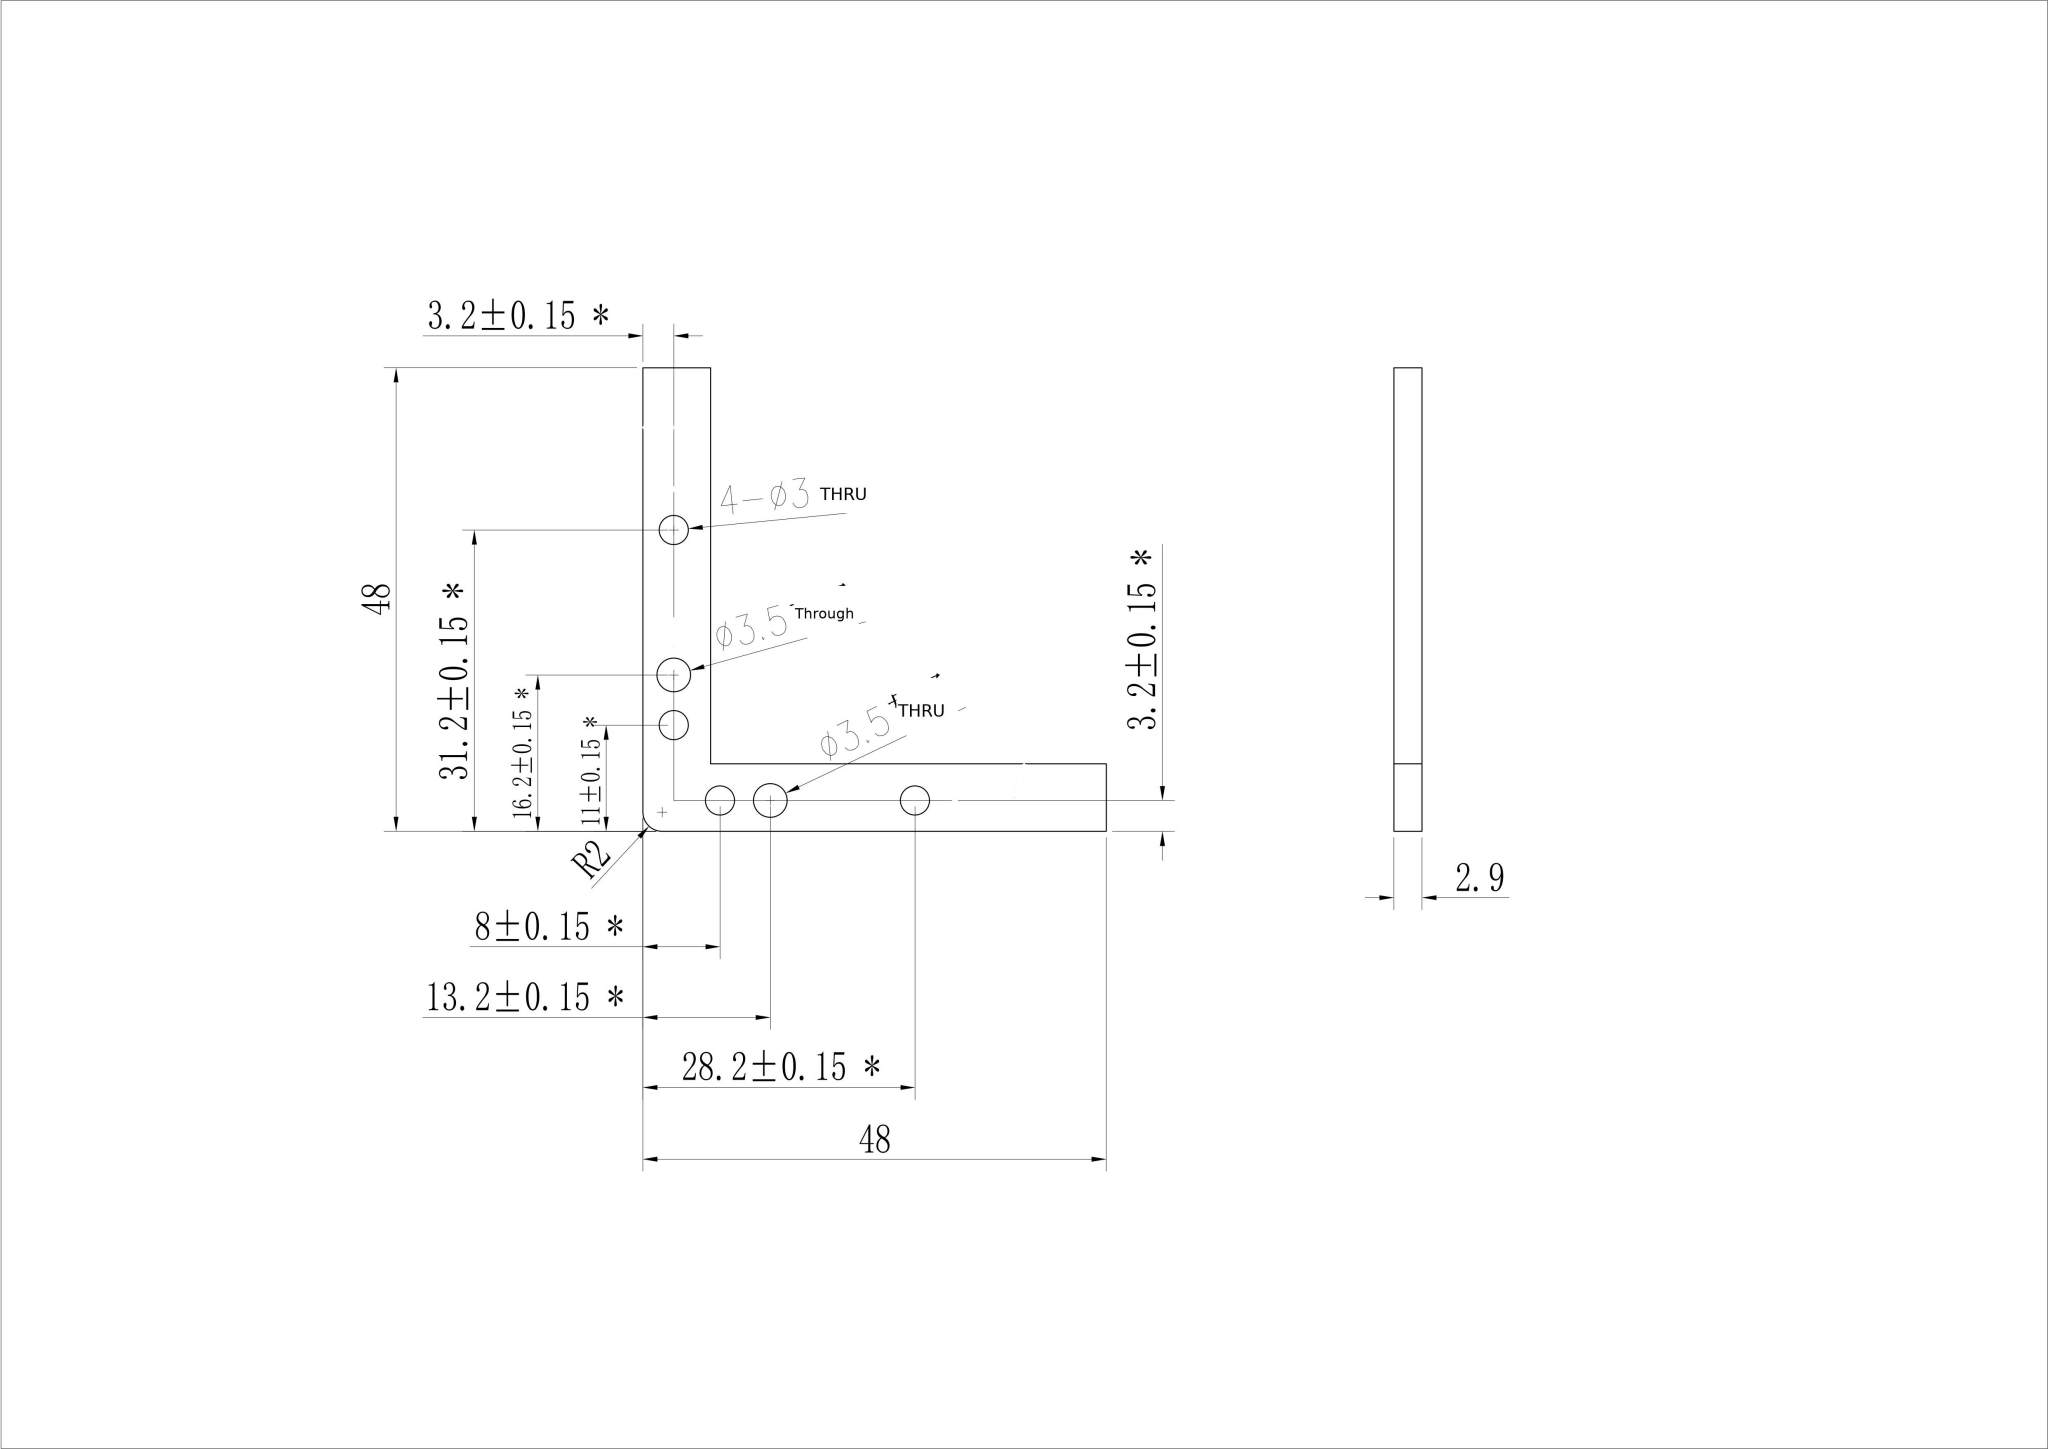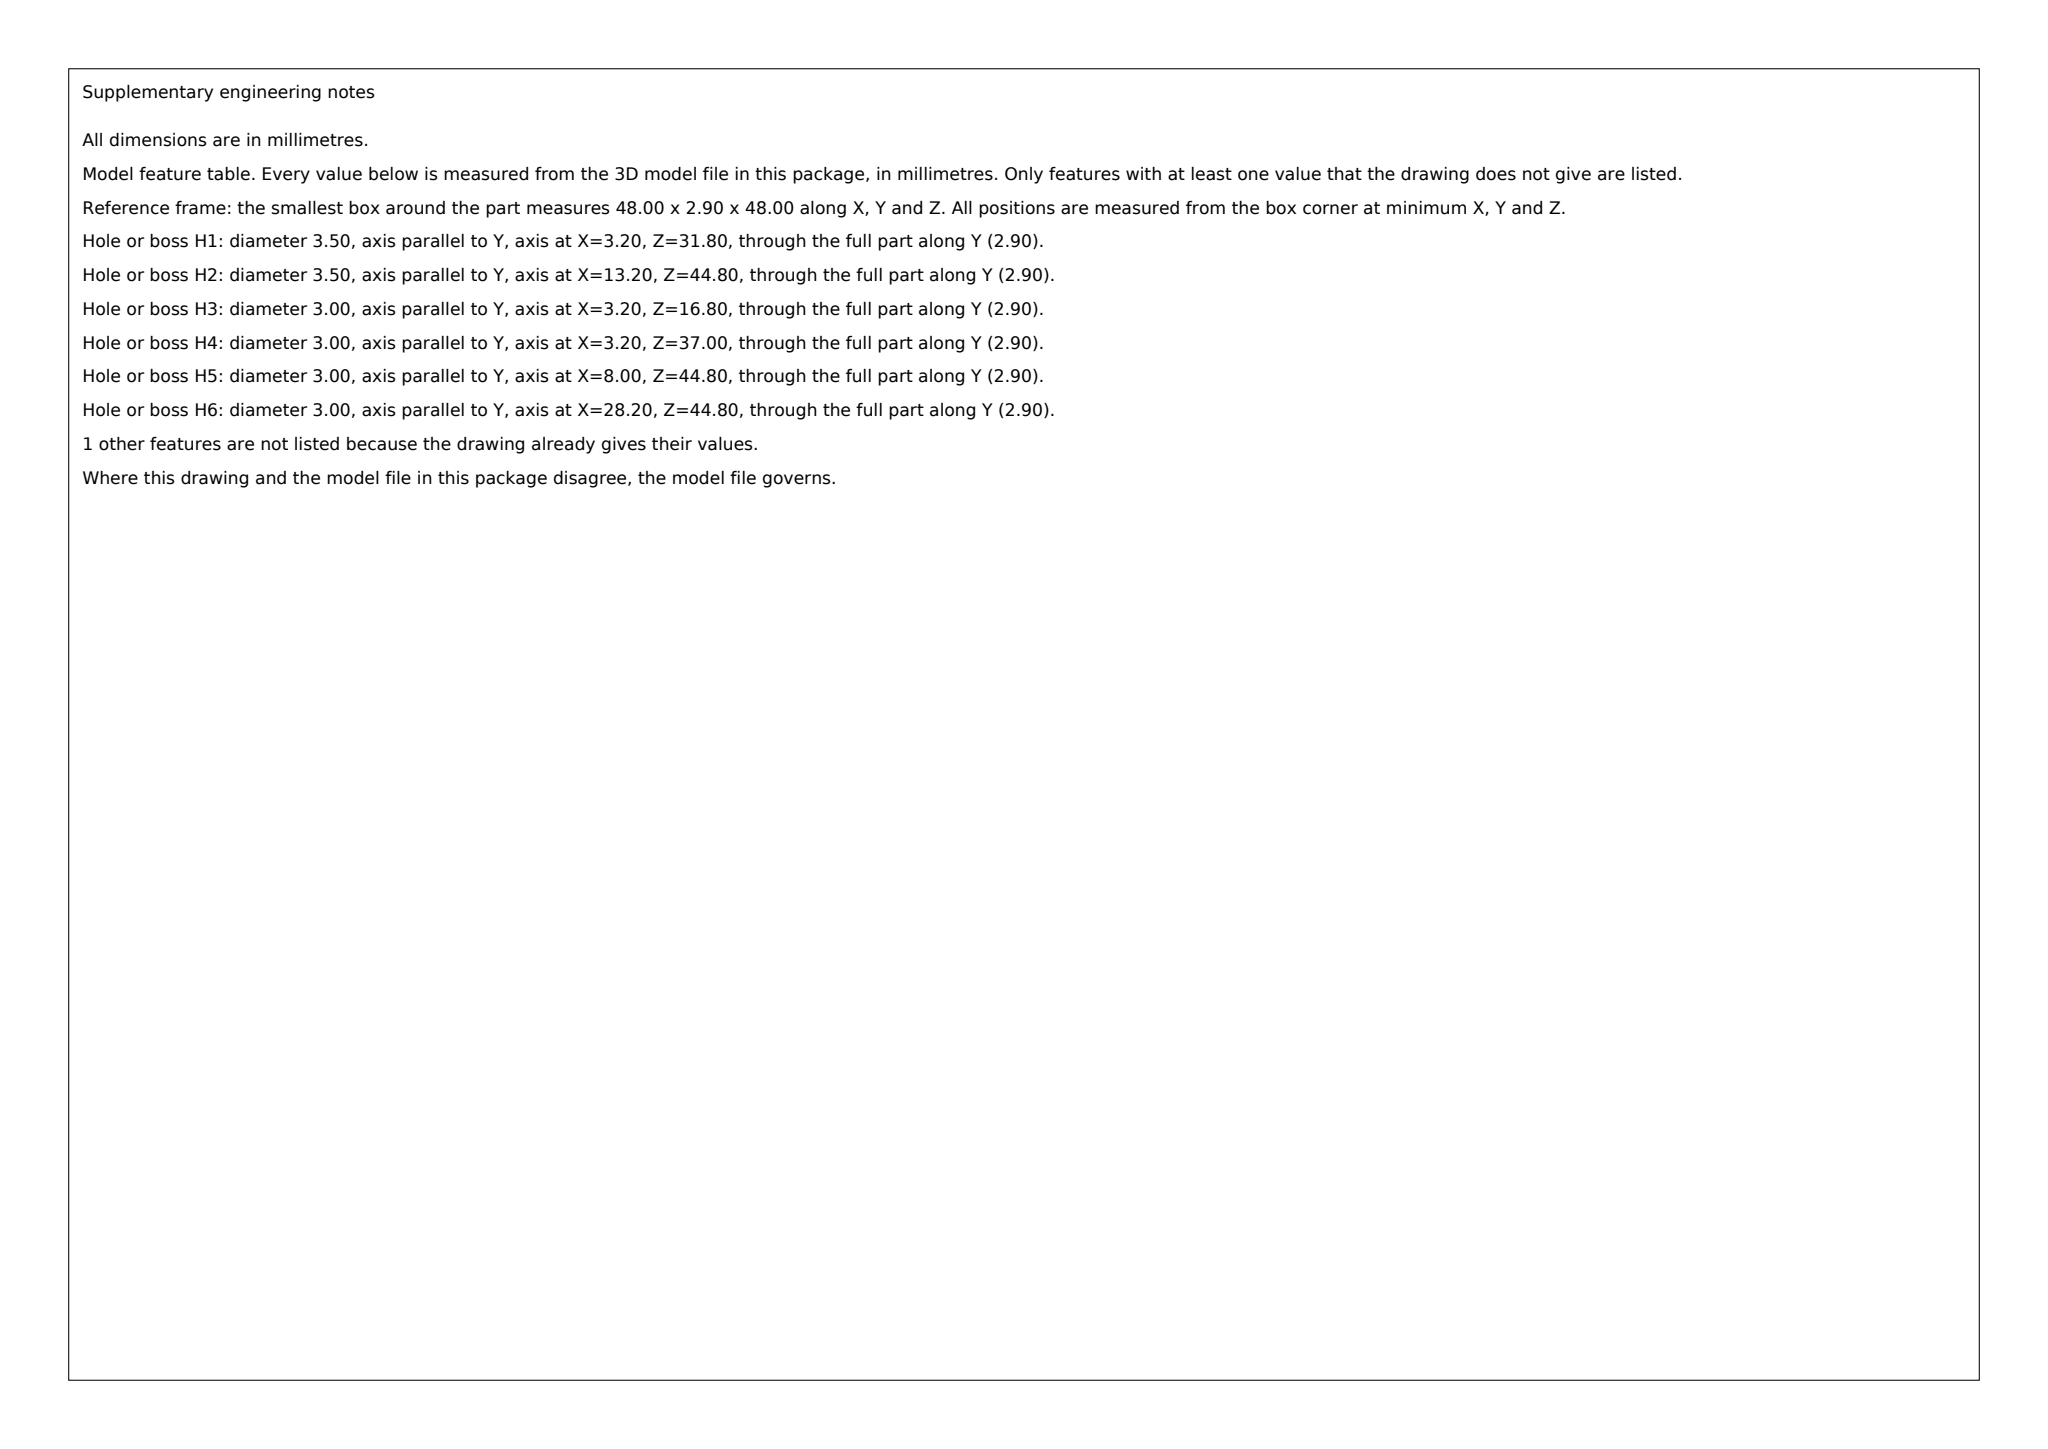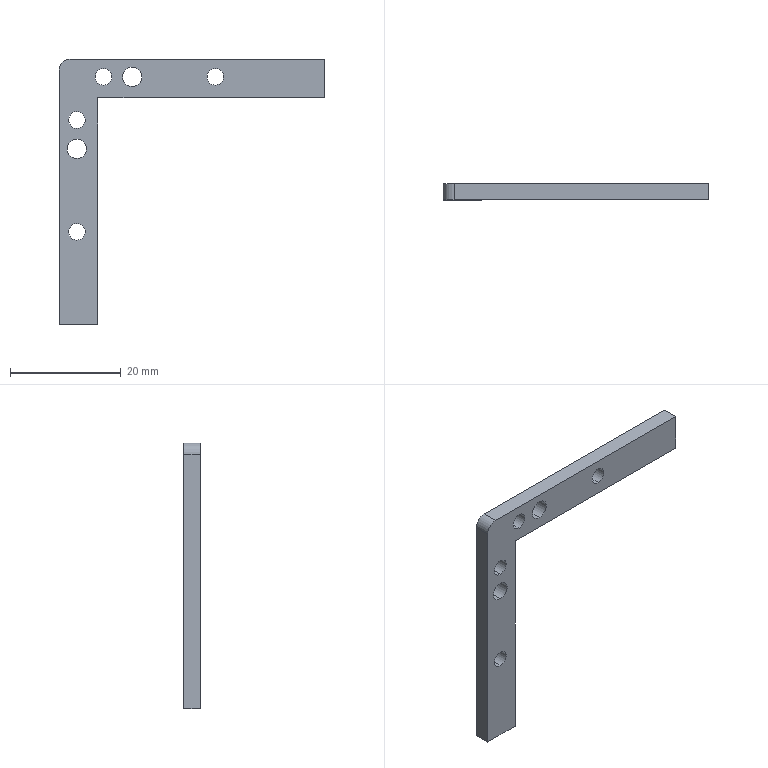Part | SolidWorks | mm | 1 solid | 21 faces | box 48 x 2.9 x 48 mm | volume 1666 mm3 | cylinder 13 | plane 8 | commonest cylinder face diameters 3 x8 3.5 x4 4 x1
STEP:
#1=CARTESIAN_POINT('',(-44.8,2.9,-29.7));
#2=VERTEX_POINT('',#1);
#3=CARTESIAN_POINT('',(-44.8,2.9,-32.7));
#4=VERTEX_POINT('',#3);
#5=CARTESIAN_POINT('',(-44.8,2.9,-31.2));
#6=DIRECTION('',(0.,-1.,0.));
#7=DIRECTION('',(0.,0.,-1.));
#8=AXIS2_PLACEMENT_3D('',#5,#6,#7);
#9=CIRCLE('',#8,1.5);
#10=EDGE_CURVE('',#2,#4,#9,.T.);
#11=ORIENTED_EDGE('',*,*,#10,.F.);
#12=CARTESIAN_POINT('',(-44.8,0.,-29.7));
#13=VERTEX_POINT('',#12);
#14=CARTESIAN_POINT('',(-44.8,2.9,-29.7));
#15=DIRECTION('',(0.,-1.,0.));
#16=VECTOR('',#15,1000.);
#17=LINE('',#14,#16);
#18=EDGE_CURVE('',#2,#13,#17,.T.);
#19=ORIENTED_EDGE('',*,*,#18,.T.);
#20=CARTESIAN_POINT('',(-44.8,0.,-32.7));
#21=VERTEX_POINT('',#20);
#22=CARTESIAN_POINT('',(-44.8,0.,-31.2));
#23=DIRECTION('',(0.,1.,0.));
#24=DIRECTION('',(0.,0.,-1.));
#25=AXIS2_PLACEMENT_3D('',#22,#23,#24);
#26=CIRCLE('',#25,1.5);
#27=EDGE_CURVE('',#21,#13,#26,.T.);
#28=ORIENTED_EDGE('',*,*,#27,.F.);
#29=CARTESIAN_POINT('',(-44.8,2.9,-32.7));
#30=DIRECTION('',(0.,-1.,0.));
#31=VECTOR('',#30,1000.);
#32=LINE('',#29,#31);
#33=EDGE_CURVE('',#4,#21,#32,.T.);
#34=ORIENTED_EDGE('',*,*,#33,.F.);
#35=EDGE_LOOP('',(#11,#19,#28,#34));
#36=FACE_OUTER_BOUND('',#35,.T.);
#37=CARTESIAN_POINT('',(-44.8,2.9,-31.2));
#38=DIRECTION('',(0.,-1.,0.));
#39=DIRECTION('',(0.,0.,-1.));
#40=AXIS2_PLACEMENT_3D('',#37,#38,#39);
#41=CYLINDRICAL_SURFACE('',#40,1.5);
#42=ADVANCED_FACE('',(#36),#41,.F.);
#43=CARTESIAN_POINT('',(-44.8,2.9,-14.45));
#44=VERTEX_POINT('',#43);
#45=CARTESIAN_POINT('',(-44.8,2.9,-17.95));
#46=VERTEX_POINT('',#45);
#47=CARTESIAN_POINT('',(-44.8,2.9,-16.2));
#48=DIRECTION('',(0.,-1.,0.));
#49=DIRECTION('',(0.,0.,-1.));
#50=AXIS2_PLACEMENT_3D('',#47,#48,#49);
#51=CIRCLE('',#50,1.75);
#52=EDGE_CURVE('',#44,#46,#51,.T.);
#53=ORIENTED_EDGE('',*,*,#52,.F.);
#54=CARTESIAN_POINT('',(-44.8,0.,-14.45));
#55=VERTEX_POINT('',#54);
#56=CARTESIAN_POINT('',(-44.8,2.9,-14.45));
#57=DIRECTION('',(0.,-1.,0.));
#58=VECTOR('',#57,1000.);
#59=LINE('',#56,#58);
#60=EDGE_CURVE('',#44,#55,#59,.T.);
#61=ORIENTED_EDGE('',*,*,#60,.T.);
#62=CARTESIAN_POINT('',(-44.8,0.,-17.95));
#63=VERTEX_POINT('',#62);
#64=CARTESIAN_POINT('',(-44.8,0.,-16.2));
#65=DIRECTION('',(0.,1.,0.));
#66=DIRECTION('',(0.,0.,-1.));
#67=AXIS2_PLACEMENT_3D('',#64,#65,#66);
#68=CIRCLE('',#67,1.75);
#69=EDGE_CURVE('',#63,#55,#68,.T.);
#70=ORIENTED_EDGE('',*,*,#69,.F.);
#71=CARTESIAN_POINT('',(-44.8,2.9,-17.95));
#72=DIRECTION('',(0.,-1.,0.));
#73=VECTOR('',#72,1000.);
#74=LINE('',#71,#73);
#75=EDGE_CURVE('',#46,#63,#74,.T.);
#76=ORIENTED_EDGE('',*,*,#75,.F.);
#77=EDGE_LOOP('',(#53,#61,#70,#76));
#78=FACE_OUTER_BOUND('',#77,.T.);
#79=CARTESIAN_POINT('',(-44.8,2.9,-16.2));
#80=DIRECTION('',(0.,-1.,0.));
#81=DIRECTION('',(0.,0.,-1.));
#82=AXIS2_PLACEMENT_3D('',#79,#80,#81);
#83=CYLINDRICAL_SURFACE('',#82,1.75);
#84=ADVANCED_FACE('',(#78),#83,.F.);
#85=CARTESIAN_POINT('',(-34.8,2.9,-1.45));
#86=VERTEX_POINT('',#85);
#87=CARTESIAN_POINT('',(-34.8,2.9,-4.95));
#88=VERTEX_POINT('',#87);
#89=CARTESIAN_POINT('',(-34.8,2.9,-3.2));
#90=DIRECTION('',(0.,-1.,0.));
#91=DIRECTION('',(0.,0.,-1.));
#92=AXIS2_PLACEMENT_3D('',#89,#90,#91);
#93=CIRCLE('',#92,1.75);
#94=EDGE_CURVE('',#86,#88,#93,.T.);
#95=ORIENTED_EDGE('',*,*,#94,.F.);
#96=CARTESIAN_POINT('',(-34.8,0.,-1.45));
#97=VERTEX_POINT('',#96);
#98=CARTESIAN_POINT('',(-34.8,2.9,-1.45));
#99=DIRECTION('',(0.,-1.,0.));
#100=VECTOR('',#99,1000.);
#101=LINE('',#98,#100);
#102=EDGE_CURVE('',#86,#97,#101,.T.);
#103=ORIENTED_EDGE('',*,*,#102,.T.);
#104=CARTESIAN_POINT('',(-34.8,0.,-4.95));
#105=VERTEX_POINT('',#104);
#106=CARTESIAN_POINT('',(-34.8,0.,-3.2));
#107=DIRECTION('',(0.,1.,0.));
#108=DIRECTION('',(0.,0.,-1.));
#109=AXIS2_PLACEMENT_3D('',#106,#107,#108);
#110=CIRCLE('',#109,1.75);
#111=EDGE_CURVE('',#105,#97,#110,.T.);
#112=ORIENTED_EDGE('',*,*,#111,.F.);
#113=CARTESIAN_POINT('',(-34.8,2.9,-4.95));
#114=DIRECTION('',(0.,-1.,0.));
#115=VECTOR('',#114,1000.);
#116=LINE('',#113,#115);
#117=EDGE_CURVE('',#88,#105,#116,.T.);
#118=ORIENTED_EDGE('',*,*,#117,.F.);
#119=EDGE_LOOP('',(#95,#103,#112,#118));
#120=FACE_OUTER_BOUND('',#119,.T.);
#121=CARTESIAN_POINT('',(-34.8,2.9,-3.2));
#122=DIRECTION('',(0.,-1.,0.));
#123=DIRECTION('',(0.,0.,-1.));
#124=AXIS2_PLACEMENT_3D('',#121,#122,#123);
#125=CYLINDRICAL_SURFACE('',#124,1.75);
#126=ADVANCED_FACE('',(#120),#125,.F.);
#127=CARTESIAN_POINT('',(-40.,2.9,-1.7));
#128=VERTEX_POINT('',#127);
#129=CARTESIAN_POINT('',(-40.,2.9,-4.7));
#130=VERTEX_POINT('',#129);
#131=CARTESIAN_POINT('',(-40.,2.9,-3.2));
#132=DIRECTION('',(0.,-1.,0.));
#133=DIRECTION('',(0.,0.,-1.));
#134=AXIS2_PLACEMENT_3D('',#131,#132,#133);
#135=CIRCLE('',#134,1.5);
#136=EDGE_CURVE('',#128,#130,#135,.T.);
#137=ORIENTED_EDGE('',*,*,#136,.F.);
#138=CARTESIAN_POINT('',(-40.,0.,-1.7));
#139=VERTEX_POINT('',#138);
#140=CARTESIAN_POINT('',(-40.,2.9,-1.7));
#141=DIRECTION('',(0.,-1.,0.));
#142=VECTOR('',#141,1000.);
#143=LINE('',#140,#142);
#144=EDGE_CURVE('',#128,#139,#143,.T.);
#145=ORIENTED_EDGE('',*,*,#144,.T.);
#146=CARTESIAN_POINT('',(-40.,0.,-4.7));
#147=VERTEX_POINT('',#146);
#148=CARTESIAN_POINT('',(-40.,0.,-3.2));
#149=DIRECTION('',(0.,1.,0.));
#150=DIRECTION('',(0.,0.,-1.));
#151=AXIS2_PLACEMENT_3D('',#148,#149,#150);
#152=CIRCLE('',#151,1.5);
#153=EDGE_CURVE('',#147,#139,#152,.T.);
#154=ORIENTED_EDGE('',*,*,#153,.F.);
#155=CARTESIAN_POINT('',(-40.,2.9,-4.7));
#156=DIRECTION('',(0.,-1.,0.));
#157=VECTOR('',#156,1000.);
#158=LINE('',#155,#157);
#159=EDGE_CURVE('',#130,#147,#158,.T.);
#160=ORIENTED_EDGE('',*,*,#159,.F.);
#161=EDGE_LOOP('',(#137,#145,#154,#160));
#162=FACE_OUTER_BOUND('',#161,.T.);
#163=CARTESIAN_POINT('',(-40.,2.9,-3.2));
#164=DIRECTION('',(0.,-1.,0.));
#165=DIRECTION('',(0.,0.,-1.));
#166=AXIS2_PLACEMENT_3D('',#163,#164,#165);
#167=CYLINDRICAL_SURFACE('',#166,1.5);
#168=ADVANCED_FACE('',(#162),#167,.F.);
#169=CARTESIAN_POINT('',(-19.8,2.9,-1.7));
#170=VERTEX_POINT('',#169);
#171=CARTESIAN_POINT('',(-19.8,2.9,-4.7));
#172=VERTEX_POINT('',#171);
#173=CARTESIAN_POINT('',(-19.8,2.9,-3.2));
#174=DIRECTION('',(0.,-1.,0.));
#175=DIRECTION('',(0.,0.,-1.));
#176=AXIS2_PLACEMENT_3D('',#173,#174,#175);
#177=CIRCLE('',#176,1.5);
#178=EDGE_CURVE('',#170,#172,#177,.T.);
#179=ORIENTED_EDGE('',*,*,#178,.F.);
#180=CARTESIAN_POINT('',(-19.8,0.,-1.7));
#181=VERTEX_POINT('',#180);
#182=CARTESIAN_POINT('',(-19.8,2.9,-1.7));
#183=DIRECTION('',(0.,-1.,0.));
#184=VECTOR('',#183,1000.);
#185=LINE('',#182,#184);
#186=EDGE_CURVE('',#170,#181,#185,.T.);
#187=ORIENTED_EDGE('',*,*,#186,.T.);
#188=CARTESIAN_POINT('',(-19.8,0.,-4.7));
#189=VERTEX_POINT('',#188);
#190=CARTESIAN_POINT('',(-19.8,0.,-3.2));
#191=DIRECTION('',(0.,1.,0.));
#192=DIRECTION('',(0.,0.,-1.));
#193=AXIS2_PLACEMENT_3D('',#190,#191,#192);
#194=CIRCLE('',#193,1.5);
#195=EDGE_CURVE('',#189,#181,#194,.T.);
#196=ORIENTED_EDGE('',*,*,#195,.F.);
#197=CARTESIAN_POINT('',(-19.8,2.9,-4.7));
#198=DIRECTION('',(0.,-1.,0.));
#199=VECTOR('',#198,1000.);
#200=LINE('',#197,#199);
#201=EDGE_CURVE('',#172,#189,#200,.T.);
#202=ORIENTED_EDGE('',*,*,#201,.F.);
#203=EDGE_LOOP('',(#179,#187,#196,#202));
#204=FACE_OUTER_BOUND('',#203,.T.);
#205=CARTESIAN_POINT('',(-19.8,2.9,-3.2));
#206=DIRECTION('',(0.,-1.,0.));
#207=DIRECTION('',(0.,0.,-1.));
#208=AXIS2_PLACEMENT_3D('',#205,#206,#207);
#209=CYLINDRICAL_SURFACE('',#208,1.5);
#210=ADVANCED_FACE('',(#204),#209,.F.);
#211=CARTESIAN_POINT('',(-44.8,2.9,-9.5));
#212=VERTEX_POINT('',#211);
#213=CARTESIAN_POINT('',(-44.8,2.9,-12.5));
#214=VERTEX_POINT('',#213);
#215=CARTESIAN_POINT('',(-44.8,2.9,-11.));
#216=DIRECTION('',(0.,-1.,0.));
#217=DIRECTION('',(0.,0.,-1.));
#218=AXIS2_PLACEMENT_3D('',#215,#216,#217);
#219=CIRCLE('',#218,1.5);
#220=EDGE_CURVE('',#212,#214,#219,.T.);
#221=ORIENTED_EDGE('',*,*,#220,.F.);
#222=CARTESIAN_POINT('',(-44.8,0.,-9.5));
#223=VERTEX_POINT('',#222);
#224=CARTESIAN_POINT('',(-44.8,2.9,-9.5));
#225=DIRECTION('',(0.,-1.,0.));
#226=VECTOR('',#225,1000.);
#227=LINE('',#224,#226);
#228=EDGE_CURVE('',#212,#223,#227,.T.);
#229=ORIENTED_EDGE('',*,*,#228,.T.);
#230=CARTESIAN_POINT('',(-44.8,0.,-12.5));
#231=VERTEX_POINT('',#230);
#232=CARTESIAN_POINT('',(-44.8,0.,-11.));
#233=DIRECTION('',(0.,1.,0.));
#234=DIRECTION('',(0.,0.,-1.));
#235=AXIS2_PLACEMENT_3D('',#232,#233,#234);
#236=CIRCLE('',#235,1.5);
#237=EDGE_CURVE('',#231,#223,#236,.T.);
#238=ORIENTED_EDGE('',*,*,#237,.F.);
#239=CARTESIAN_POINT('',(-44.8,2.9,-12.5));
#240=DIRECTION('',(0.,-1.,0.));
#241=VECTOR('',#240,1000.);
#242=LINE('',#239,#241);
#243=EDGE_CURVE('',#214,#231,#242,.T.);
#244=ORIENTED_EDGE('',*,*,#243,.F.);
#245=EDGE_LOOP('',(#221,#229,#238,#244));
#246=FACE_OUTER_BOUND('',#245,.T.);
#247=CARTESIAN_POINT('',(-44.8,2.9,-11.));
#248=DIRECTION('',(0.,-1.,0.));
#249=DIRECTION('',(0.,0.,-1.));
#250=AXIS2_PLACEMENT_3D('',#247,#248,#249);
#251=CYLINDRICAL_SURFACE('',#250,1.5);
#252=ADVANCED_FACE('',(#246),#251,.F.);
#253=CARTESIAN_POINT('',(-44.8,2.9,-31.2));
#254=DIRECTION('',(0.,-1.,0.));
#255=DIRECTION('',(0.,0.,-1.));
#256=AXIS2_PLACEMENT_3D('',#253,#254,#255);
#257=CIRCLE('',#256,1.5);
#258=EDGE_CURVE('',#4,#2,#257,.T.);
#259=ORIENTED_EDGE('',*,*,#258,.T.);
#260=ORIENTED_EDGE('',*,*,#10,.T.);
#261=EDGE_LOOP('',(#259,#260));
#262=FACE_BOUND('',#261,.T.);
#263=CARTESIAN_POINT('',(-44.8,2.9,-16.2));
#264=DIRECTION('',(0.,-1.,0.));
#265=DIRECTION('',(0.,0.,-1.));
#266=AXIS2_PLACEMENT_3D('',#263,#264,#265);
#267=CIRCLE('',#266,1.75);
#268=EDGE_CURVE('',#46,#44,#267,.T.);
#269=ORIENTED_EDGE('',*,*,#268,.T.);
#270=ORIENTED_EDGE('',*,*,#52,.T.);
#271=EDGE_LOOP('',(#269,#270));
#272=FACE_BOUND('',#271,.T.);
#273=CARTESIAN_POINT('',(-34.8,2.9,-3.2));
#274=DIRECTION('',(0.,-1.,0.));
#275=DIRECTION('',(0.,0.,-1.));
#276=AXIS2_PLACEMENT_3D('',#273,#274,#275);
#277=CIRCLE('',#276,1.75);
#278=EDGE_CURVE('',#88,#86,#277,.T.);
#279=ORIENTED_EDGE('',*,*,#278,.T.);
#280=ORIENTED_EDGE('',*,*,#94,.T.);
#281=EDGE_LOOP('',(#279,#280));
#282=FACE_BOUND('',#281,.T.);
#283=CARTESIAN_POINT('',(0.,2.9,-7.));
#284=VERTEX_POINT('',#283);
#285=CARTESIAN_POINT('',(-41.,2.9,-7.));
#286=VERTEX_POINT('',#285);
#287=CARTESIAN_POINT('',(-46.,2.9,-7.));
#288=DIRECTION('',(-1.,0.,0.));
#289=VECTOR('',#288,1000.);
#290=LINE('',#287,#289);
#291=EDGE_CURVE('',#284,#286,#290,.T.);
#292=ORIENTED_EDGE('',*,*,#291,.T.);
#293=CARTESIAN_POINT('',(-41.,2.9,-48.));
#294=VERTEX_POINT('',#293);
#295=CARTESIAN_POINT('',(-41.,2.9,-2.));
#296=DIRECTION('',(0.,0.,-1.));
#297=VECTOR('',#296,1000.);
#298=LINE('',#295,#297);
#299=EDGE_CURVE('',#286,#294,#298,.T.);
#300=ORIENTED_EDGE('',*,*,#299,.T.);
#301=CARTESIAN_POINT('',(-48.,2.9,-48.));
#302=VERTEX_POINT('',#301);
#303=CARTESIAN_POINT('',(-46.,2.9,-48.));
#304=DIRECTION('',(-1.,0.,0.));
#305=VECTOR('',#304,1000.);
#306=LINE('',#303,#305);
#307=EDGE_CURVE('',#294,#302,#306,.T.);
#308=ORIENTED_EDGE('',*,*,#307,.T.);
#309=CARTESIAN_POINT('',(-48.,2.9,-2.));
#310=VERTEX_POINT('',#309);
#311=CARTESIAN_POINT('',(-48.,2.9,-2.));
#312=DIRECTION('',(0.,0.,1.));
#313=VECTOR('',#312,1000.);
#314=LINE('',#311,#313);
#315=EDGE_CURVE('',#302,#310,#314,.T.);
#316=ORIENTED_EDGE('',*,*,#315,.T.);
#317=CARTESIAN_POINT('',(-46.,2.9,0.));
#318=VERTEX_POINT('',#317);
#319=CARTESIAN_POINT('',(-46.,2.9,-2.));
#320=DIRECTION('',(0.,1.,0.));
#321=DIRECTION('',(0.,0.,-1.));
#322=AXIS2_PLACEMENT_3D('',#319,#320,#321);
#323=CIRCLE('',#322,2.);
#324=EDGE_CURVE('',#310,#318,#323,.T.);
#325=ORIENTED_EDGE('',*,*,#324,.T.);
#326=CARTESIAN_POINT('',(0.,2.9,0.));
#327=VERTEX_POINT('',#326);
#328=CARTESIAN_POINT('',(-46.,2.9,0.));
#329=DIRECTION('',(1.,0.,0.));
#330=VECTOR('',#329,1000.);
#331=LINE('',#328,#330);
#332=EDGE_CURVE('',#318,#327,#331,.T.);
#333=ORIENTED_EDGE('',*,*,#332,.T.);
#334=CARTESIAN_POINT('',(0.,2.9,-2.));
#335=DIRECTION('',(0.,0.,-1.));
#336=VECTOR('',#335,1000.);
#337=LINE('',#334,#336);
#338=EDGE_CURVE('',#327,#284,#337,.T.);
#339=ORIENTED_EDGE('',*,*,#338,.T.);
#340=EDGE_LOOP('',(#292,#300,#308,#316,#325,#333,#339));
#341=FACE_OUTER_BOUND('',#340,.T.);
#342=CARTESIAN_POINT('',(-40.,2.9,-3.2));
#343=DIRECTION('',(0.,-1.,0.));
#344=DIRECTION('',(0.,0.,-1.));
#345=AXIS2_PLACEMENT_3D('',#342,#343,#344);
#346=CIRCLE('',#345,1.5);
#347=EDGE_CURVE('',#130,#128,#346,.T.);
#348=ORIENTED_EDGE('',*,*,#347,.T.);
#349=ORIENTED_EDGE('',*,*,#136,.T.);
#350=EDGE_LOOP('',(#348,#349));
#351=FACE_BOUND('',#350,.T.);
#352=CARTESIAN_POINT('',(-19.8,2.9,-3.2));
#353=DIRECTION('',(0.,-1.,0.));
#354=DIRECTION('',(0.,0.,-1.));
#355=AXIS2_PLACEMENT_3D('',#352,#353,#354);
#356=CIRCLE('',#355,1.5);
#357=EDGE_CURVE('',#172,#170,#356,.T.);
#358=ORIENTED_EDGE('',*,*,#357,.T.);
#359=ORIENTED_EDGE('',*,*,#178,.T.);
#360=EDGE_LOOP('',(#358,#359));
#361=FACE_BOUND('',#360,.T.);
#362=CARTESIAN_POINT('',(-44.8,2.9,-11.));
#363=DIRECTION('',(0.,-1.,0.));
#364=DIRECTION('',(0.,0.,-1.));
#365=AXIS2_PLACEMENT_3D('',#362,#363,#364);
#366=CIRCLE('',#365,1.5);
#367=EDGE_CURVE('',#214,#212,#366,.T.);
#368=ORIENTED_EDGE('',*,*,#367,.T.);
#369=ORIENTED_EDGE('',*,*,#220,.T.);
#370=EDGE_LOOP('',(#368,#369));
#371=FACE_BOUND('',#370,.T.);
#372=CARTESIAN_POINT('',(-46.,2.9,-2.));
#373=DIRECTION('',(0.,1.,0.));
#374=DIRECTION('',(0.,0.,1.));
#375=AXIS2_PLACEMENT_3D('',#372,#373,#374);
#376=PLANE('',#375);
#377=ADVANCED_FACE('',(#262,#272,#282,#341,#351,#361,#371),#376,.T.);
#378=ORIENTED_EDGE('',*,*,#18,.F.);
#379=ORIENTED_EDGE('',*,*,#258,.F.);
#380=ORIENTED_EDGE('',*,*,#33,.T.);
#381=CARTESIAN_POINT('',(-44.8,0.,-31.2));
#382=DIRECTION('',(0.,1.,0.));
#383=DIRECTION('',(0.,0.,-1.));
#384=AXIS2_PLACEMENT_3D('',#381,#382,#383);
#385=CIRCLE('',#384,1.5);
#386=EDGE_CURVE('',#13,#21,#385,.T.);
#387=ORIENTED_EDGE('',*,*,#386,.F.);
#388=EDGE_LOOP('',(#378,#379,#380,#387));
#389=FACE_OUTER_BOUND('',#388,.T.);
#390=CARTESIAN_POINT('',(-44.8,2.9,-31.2));
#391=DIRECTION('',(0.,-1.,0.));
#392=DIRECTION('',(0.,0.,-1.));
#393=AXIS2_PLACEMENT_3D('',#390,#391,#392);
#394=CYLINDRICAL_SURFACE('',#393,1.5);
#395=ADVANCED_FACE('',(#389),#394,.F.);
#396=ORIENTED_EDGE('',*,*,#60,.F.);
#397=ORIENTED_EDGE('',*,*,#268,.F.);
#398=ORIENTED_EDGE('',*,*,#75,.T.);
#399=CARTESIAN_POINT('',(-44.8,0.,-16.2));
#400=DIRECTION('',(0.,1.,0.));
#401=DIRECTION('',(0.,0.,-1.));
#402=AXIS2_PLACEMENT_3D('',#399,#400,#401);
#403=CIRCLE('',#402,1.75);
#404=EDGE_CURVE('',#55,#63,#403,.T.);
#405=ORIENTED_EDGE('',*,*,#404,.F.);
#406=EDGE_LOOP('',(#396,#397,#398,#405));
#407=FACE_OUTER_BOUND('',#406,.T.);
#408=CARTESIAN_POINT('',(-44.8,2.9,-16.2));
#409=DIRECTION('',(0.,-1.,0.));
#410=DIRECTION('',(0.,0.,-1.));
#411=AXIS2_PLACEMENT_3D('',#408,#409,#410);
#412=CYLINDRICAL_SURFACE('',#411,1.75);
#413=ADVANCED_FACE('',(#407),#412,.F.);
#414=ORIENTED_EDGE('',*,*,#102,.F.);
#415=ORIENTED_EDGE('',*,*,#278,.F.);
#416=ORIENTED_EDGE('',*,*,#117,.T.);
#417=CARTESIAN_POINT('',(-34.8,0.,-3.2));
#418=DIRECTION('',(0.,1.,0.));
#419=DIRECTION('',(0.,0.,-1.));
#420=AXIS2_PLACEMENT_3D('',#417,#418,#419);
#421=CIRCLE('',#420,1.75);
#422=EDGE_CURVE('',#97,#105,#421,.T.);
#423=ORIENTED_EDGE('',*,*,#422,.F.);
#424=EDGE_LOOP('',(#414,#415,#416,#423));
#425=FACE_OUTER_BOUND('',#424,.T.);
#426=CARTESIAN_POINT('',(-34.8,2.9,-3.2));
#427=DIRECTION('',(0.,-1.,0.));
#428=DIRECTION('',(0.,0.,-1.));
#429=AXIS2_PLACEMENT_3D('',#426,#427,#428);
#430=CYLINDRICAL_SURFACE('',#429,1.75);
#431=ADVANCED_FACE('',(#425),#430,.F.);
#432=CARTESIAN_POINT('',(-41.,0.,-48.));
#433=VERTEX_POINT('',#432);
#434=CARTESIAN_POINT('',(-41.,2.9,-48.));
#435=DIRECTION('',(0.,-1.,0.));
#436=VECTOR('',#435,1000.);
#437=LINE('',#434,#436);
#438=EDGE_CURVE('',#294,#433,#437,.T.);
#439=ORIENTED_EDGE('',*,*,#438,.F.);
#440=ORIENTED_EDGE('',*,*,#299,.F.);
#441=CARTESIAN_POINT('',(-41.,0.,-7.));
#442=VERTEX_POINT('',#441);
#443=CARTESIAN_POINT('',(-41.,2.9,-7.));
#444=DIRECTION('',(0.,1.,0.));
#445=VECTOR('',#444,1000.);
#446=LINE('',#443,#445);
#447=EDGE_CURVE('',#442,#286,#446,.T.);
#448=ORIENTED_EDGE('',*,*,#447,.F.);
#449=CARTESIAN_POINT('',(-41.,0.,-48.));
#450=DIRECTION('',(0.,0.,1.));
#451=VECTOR('',#450,1000.);
#452=LINE('',#449,#451);
#453=EDGE_CURVE('',#433,#442,#452,.T.);
#454=ORIENTED_EDGE('',*,*,#453,.F.);
#455=EDGE_LOOP('',(#439,#440,#448,#454));
#456=FACE_OUTER_BOUND('',#455,.T.);
#457=CARTESIAN_POINT('',(-41.,2.9,-48.));
#458=DIRECTION('',(-1.,0.,0.));
#459=DIRECTION('',(0.,0.,1.));
#460=AXIS2_PLACEMENT_3D('',#457,#458,#459);
#461=PLANE('',#460);
#462=ADVANCED_FACE('',(#456),#461,.F.);
#463=ORIENTED_EDGE('',*,*,#447,.T.);
#464=ORIENTED_EDGE('',*,*,#291,.F.);
#465=CARTESIAN_POINT('',(0.,0.,-7.));
#466=VERTEX_POINT('',#465);
#467=CARTESIAN_POINT('',(0.,2.9,-7.));
#468=DIRECTION('',(0.,1.,0.));
#469=VECTOR('',#468,1000.);
#470=LINE('',#467,#469);
#471=EDGE_CURVE('',#466,#284,#470,.T.);
#472=ORIENTED_EDGE('',*,*,#471,.F.);
#473=CARTESIAN_POINT('',(-41.,0.,-7.));
#474=DIRECTION('',(1.,0.,0.));
#475=VECTOR('',#474,1000.);
#476=LINE('',#473,#475);
#477=EDGE_CURVE('',#442,#466,#476,.T.);
#478=ORIENTED_EDGE('',*,*,#477,.F.);
#479=EDGE_LOOP('',(#463,#464,#472,#478));
#480=FACE_OUTER_BOUND('',#479,.T.);
#481=CARTESIAN_POINT('',(-41.,2.9,-7.));
#482=DIRECTION('',(0.,0.,1.));
#483=DIRECTION('',(1.,0.,0.));
#484=AXIS2_PLACEMENT_3D('',#481,#482,#483);
#485=PLANE('',#484);
#486=ADVANCED_FACE('',(#480),#485,.F.);
#487=ORIENTED_EDGE('',*,*,#471,.T.);
#488=ORIENTED_EDGE('',*,*,#338,.F.);
#489=CARTESIAN_POINT('',(0.,0.,0.));
#490=VERTEX_POINT('',#489);
#491=CARTESIAN_POINT('',(0.,2.9,0.));
#492=DIRECTION('',(0.,1.,0.));
#493=VECTOR('',#492,1000.);
#494=LINE('',#491,#493);
#495=EDGE_CURVE('',#490,#327,#494,.T.);
#496=ORIENTED_EDGE('',*,*,#495,.F.);
#497=CARTESIAN_POINT('',(0.,0.,-7.));
#498=DIRECTION('',(0.,0.,1.));
#499=VECTOR('',#498,1000.);
#500=LINE('',#497,#499);
#501=EDGE_CURVE('',#466,#490,#500,.T.);
#502=ORIENTED_EDGE('',*,*,#501,.F.);
#503=EDGE_LOOP('',(#487,#488,#496,#502));
#504=FACE_OUTER_BOUND('',#503,.T.);
#505=CARTESIAN_POINT('',(0.,2.9,-7.));
#506=DIRECTION('',(-1.,0.,0.));
#507=DIRECTION('',(0.,0.,1.));
#508=AXIS2_PLACEMENT_3D('',#505,#506,#507);
#509=PLANE('',#508);
#510=ADVANCED_FACE('',(#504),#509,.F.);
#511=ORIENTED_EDGE('',*,*,#495,.T.);
#512=ORIENTED_EDGE('',*,*,#332,.F.);
#513=CARTESIAN_POINT('',(-46.,0.,0.));
#514=VERTEX_POINT('',#513);
#515=CARTESIAN_POINT('',(-46.,2.9,0.));
#516=DIRECTION('',(0.,1.,0.));
#517=VECTOR('',#516,1000.);
#518=LINE('',#515,#517);
#519=EDGE_CURVE('',#514,#318,#518,.T.);
#520=ORIENTED_EDGE('',*,*,#519,.F.);
#521=CARTESIAN_POINT('',(0.,0.,0.));
#522=DIRECTION('',(-1.,0.,0.));
#523=VECTOR('',#522,1000.);
#524=LINE('',#521,#523);
#525=EDGE_CURVE('',#490,#514,#524,.T.);
#526=ORIENTED_EDGE('',*,*,#525,.F.);
#527=EDGE_LOOP('',(#511,#512,#520,#526));
#528=FACE_OUTER_BOUND('',#527,.T.);
#529=CARTESIAN_POINT('',(0.,2.9,0.));
#530=DIRECTION('',(0.,0.,-1.));
#531=DIRECTION('',(-1.,0.,0.));
#532=AXIS2_PLACEMENT_3D('',#529,#530,#531);
#533=PLANE('',#532);
#534=ADVANCED_FACE('',(#528),#533,.F.);
#535=ORIENTED_EDGE('',*,*,#324,.F.);
#536=CARTESIAN_POINT('',(-48.,0.,-2.));
#537=VERTEX_POINT('',#536);
#538=CARTESIAN_POINT('',(-48.,2.9,-2.));
#539=DIRECTION('',(0.,-1.,0.));
#540=VECTOR('',#539,1000.);
#541=LINE('',#538,#540);
#542=EDGE_CURVE('',#310,#537,#541,.T.);
#543=ORIENTED_EDGE('',*,*,#542,.T.);
#544=CARTESIAN_POINT('',(-46.,0.,-2.));
#545=DIRECTION('',(0.,1.,0.));
#546=DIRECTION('',(0.,0.,-1.));
#547=AXIS2_PLACEMENT_3D('',#544,#545,#546);
#548=CIRCLE('',#547,2.);
#549=EDGE_CURVE('',#537,#514,#548,.T.);
#550=ORIENTED_EDGE('',*,*,#549,.T.);
#551=ORIENTED_EDGE('',*,*,#519,.T.);
#552=EDGE_LOOP('',(#535,#543,#550,#551));
#553=FACE_OUTER_BOUND('',#552,.T.);
#554=CARTESIAN_POINT('',(-46.,2.9,-2.));
#555=DIRECTION('',(0.,-1.,0.));
#556=DIRECTION('',(0.,0.,-1.));
#557=AXIS2_PLACEMENT_3D('',#554,#555,#556);
#558=CYLINDRICAL_SURFACE('',#557,2.);
#559=ADVANCED_FACE('',(#553),#558,.T.);
#560=ORIENTED_EDGE('',*,*,#542,.F.);
#561=ORIENTED_EDGE('',*,*,#315,.F.);
#562=CARTESIAN_POINT('',(-48.,0.,-48.));
#563=VERTEX_POINT('',#562);
#564=CARTESIAN_POINT('',(-48.,2.9,-48.));
#565=DIRECTION('',(0.,1.,0.));
#566=VECTOR('',#565,1000.);
#567=LINE('',#564,#566);
#568=EDGE_CURVE('',#563,#302,#567,.T.);
#569=ORIENTED_EDGE('',*,*,#568,.F.);
#570=CARTESIAN_POINT('',(-48.,0.,-2.));
#571=DIRECTION('',(0.,0.,-1.));
#572=VECTOR('',#571,1000.);
#573=LINE('',#570,#572);
#574=EDGE_CURVE('',#537,#563,#573,.T.);
#575=ORIENTED_EDGE('',*,*,#574,.F.);
#576=EDGE_LOOP('',(#560,#561,#569,#575));
#577=FACE_OUTER_BOUND('',#576,.T.);
#578=CARTESIAN_POINT('',(-48.,2.9,-2.));
#579=DIRECTION('',(1.,0.,0.));
#580=DIRECTION('',(0.,0.,-1.));
#581=AXIS2_PLACEMENT_3D('',#578,#579,#580);
#582=PLANE('',#581);
#583=ADVANCED_FACE('',(#577),#582,.F.);
#584=ORIENTED_EDGE('',*,*,#568,.T.);
#585=ORIENTED_EDGE('',*,*,#307,.F.);
#586=ORIENTED_EDGE('',*,*,#438,.T.);
#587=CARTESIAN_POINT('',(-48.,0.,-48.));
#588=DIRECTION('',(1.,0.,0.));
#589=VECTOR('',#588,1000.);
#590=LINE('',#587,#589);
#591=EDGE_CURVE('',#563,#433,#590,.T.);
#592=ORIENTED_EDGE('',*,*,#591,.F.);
#593=EDGE_LOOP('',(#584,#585,#586,#592));
#594=FACE_OUTER_BOUND('',#593,.T.);
#595=CARTESIAN_POINT('',(-48.,2.9,-48.));
#596=DIRECTION('',(0.,0.,1.));
#597=DIRECTION('',(1.,0.,0.));
#598=AXIS2_PLACEMENT_3D('',#595,#596,#597);
#599=PLANE('',#598);
#600=ADVANCED_FACE('',(#594),#599,.F.);
#601=ORIENTED_EDGE('',*,*,#144,.F.);
#602=ORIENTED_EDGE('',*,*,#347,.F.);
#603=ORIENTED_EDGE('',*,*,#159,.T.);
#604=CARTESIAN_POINT('',(-40.,0.,-3.2));
#605=DIRECTION('',(0.,1.,0.));
#606=DIRECTION('',(0.,0.,-1.));
#607=AXIS2_PLACEMENT_3D('',#604,#605,#606);
#608=CIRCLE('',#607,1.5);
#609=EDGE_CURVE('',#139,#147,#608,.T.);
#610=ORIENTED_EDGE('',*,*,#609,.F.);
#611=EDGE_LOOP('',(#601,#602,#603,#610));
#612=FACE_OUTER_BOUND('',#611,.T.);
#613=CARTESIAN_POINT('',(-40.,2.9,-3.2));
#614=DIRECTION('',(0.,-1.,0.));
#615=DIRECTION('',(0.,0.,-1.));
#616=AXIS2_PLACEMENT_3D('',#613,#614,#615);
#617=CYLINDRICAL_SURFACE('',#616,1.5);
#618=ADVANCED_FACE('',(#612),#617,.F.);
#619=ORIENTED_EDGE('',*,*,#186,.F.);
#620=ORIENTED_EDGE('',*,*,#357,.F.);
#621=ORIENTED_EDGE('',*,*,#201,.T.);
#622=CARTESIAN_POINT('',(-19.8,0.,-3.2));
#623=DIRECTION('',(0.,1.,0.));
#624=DIRECTION('',(0.,0.,-1.));
#625=AXIS2_PLACEMENT_3D('',#622,#623,#624);
#626=CIRCLE('',#625,1.5);
#627=EDGE_CURVE('',#181,#189,#626,.T.);
#628=ORIENTED_EDGE('',*,*,#627,.F.);
#629=EDGE_LOOP('',(#619,#620,#621,#628));
#630=FACE_OUTER_BOUND('',#629,.T.);
#631=CARTESIAN_POINT('',(-19.8,2.9,-3.2));
#632=DIRECTION('',(0.,-1.,0.));
#633=DIRECTION('',(0.,0.,-1.));
#634=AXIS2_PLACEMENT_3D('',#631,#632,#633);
#635=CYLINDRICAL_SURFACE('',#634,1.5);
#636=ADVANCED_FACE('',(#630),#635,.F.);
#637=ORIENTED_EDGE('',*,*,#228,.F.);
#638=ORIENTED_EDGE('',*,*,#367,.F.);
#639=ORIENTED_EDGE('',*,*,#243,.T.);
#640=CARTESIAN_POINT('',(-44.8,0.,-11.));
#641=DIRECTION('',(0.,1.,0.));
#642=DIRECTION('',(0.,0.,-1.));
#643=AXIS2_PLACEMENT_3D('',#640,#641,#642);
#644=CIRCLE('',#643,1.5);
#645=EDGE_CURVE('',#223,#231,#644,.T.);
#646=ORIENTED_EDGE('',*,*,#645,.F.);
#647=EDGE_LOOP('',(#637,#638,#639,#646));
#648=FACE_OUTER_BOUND('',#647,.T.);
#649=CARTESIAN_POINT('',(-44.8,2.9,-11.));
#650=DIRECTION('',(0.,-1.,0.));
#651=DIRECTION('',(0.,0.,-1.));
#652=AXIS2_PLACEMENT_3D('',#649,#650,#651);
#653=CYLINDRICAL_SURFACE('',#652,1.5);
#654=ADVANCED_FACE('',(#648),#653,.F.);
#655=ORIENTED_EDGE('',*,*,#27,.T.);
#656=ORIENTED_EDGE('',*,*,#386,.T.);
#657=EDGE_LOOP('',(#655,#656));
#658=FACE_BOUND('',#657,.T.);
#659=ORIENTED_EDGE('',*,*,#237,.T.);
#660=ORIENTED_EDGE('',*,*,#645,.T.);
#661=EDGE_LOOP('',(#659,#660));
#662=FACE_BOUND('',#661,.T.);
#663=ORIENTED_EDGE('',*,*,#69,.T.);
#664=ORIENTED_EDGE('',*,*,#404,.T.);
#665=EDGE_LOOP('',(#663,#664));
#666=FACE_BOUND('',#665,.T.);
#667=ORIENTED_EDGE('',*,*,#195,.T.);
#668=ORIENTED_EDGE('',*,*,#627,.T.);
#669=EDGE_LOOP('',(#667,#668));
#670=FACE_BOUND('',#669,.T.);
#671=ORIENTED_EDGE('',*,*,#111,.T.);
#672=ORIENTED_EDGE('',*,*,#422,.T.);
#673=EDGE_LOOP('',(#671,#672));
#674=FACE_BOUND('',#673,.T.);
#675=ORIENTED_EDGE('',*,*,#153,.T.);
#676=ORIENTED_EDGE('',*,*,#609,.T.);
#677=EDGE_LOOP('',(#675,#676));
#678=FACE_BOUND('',#677,.T.);
#679=ORIENTED_EDGE('',*,*,#453,.T.);
#680=ORIENTED_EDGE('',*,*,#477,.T.);
#681=ORIENTED_EDGE('',*,*,#501,.T.);
#682=ORIENTED_EDGE('',*,*,#525,.T.);
#683=ORIENTED_EDGE('',*,*,#549,.F.);
#684=ORIENTED_EDGE('',*,*,#574,.T.);
#685=ORIENTED_EDGE('',*,*,#591,.T.);
#686=EDGE_LOOP('',(#679,#680,#681,#682,#683,#684,#685));
#687=FACE_OUTER_BOUND('',#686,.T.);
#688=CARTESIAN_POINT('',(-46.,0.,-2.));
#689=DIRECTION('',(0.,1.,0.));
#690=DIRECTION('',(0.,0.,1.));
#691=AXIS2_PLACEMENT_3D('',#688,#689,#690);
#692=PLANE('',#691);
#693=ADVANCED_FACE('',(#658,#662,#666,#670,#674,#678,#687),#692,.F.);
#694=CLOSED_SHELL('',(#42,#84,#126,#168,#210,#252,#377,#395,#413,#431,#462,#486,#510,#534,#559,#583,#600,#618,#636,#654,#693));
#695=MANIFOLD_SOLID_BREP('',#694);
#696=CARTESIAN_POINT('',(0.,0.,0.));
#697=DIRECTION('',(0.,0.,1.));
#698=DIRECTION('',(1.,0.,0.));
#699=AXIS2_PLACEMENT_3D('',#696,#697,#698);
#700=(LENGTH_UNIT()NAMED_UNIT(*)SI_UNIT(.MILLI.,.METRE.));
#701=UNCERTAINTY_MEASURE_WITH_UNIT(LENGTH_MEASURE(0.00001),#700,'','');
#702=(NAMED_UNIT(*)PLANE_ANGLE_UNIT()SI_UNIT($,.RADIAN.));
#703=(NAMED_UNIT(*)SI_UNIT($,.STERADIAN.)SOLID_ANGLE_UNIT());
#704=(GEOMETRIC_REPRESENTATION_CONTEXT(3)GLOBAL_UNCERTAINTY_ASSIGNED_CONTEXT((#701))GLOBAL_UNIT_ASSIGNED_CONTEXT((#700,#702,#703))REPRESENTATION_CONTEXT('',''));
#705=ADVANCED_BREP_SHAPE_REPRESENTATION('',(#695,#699),#704);